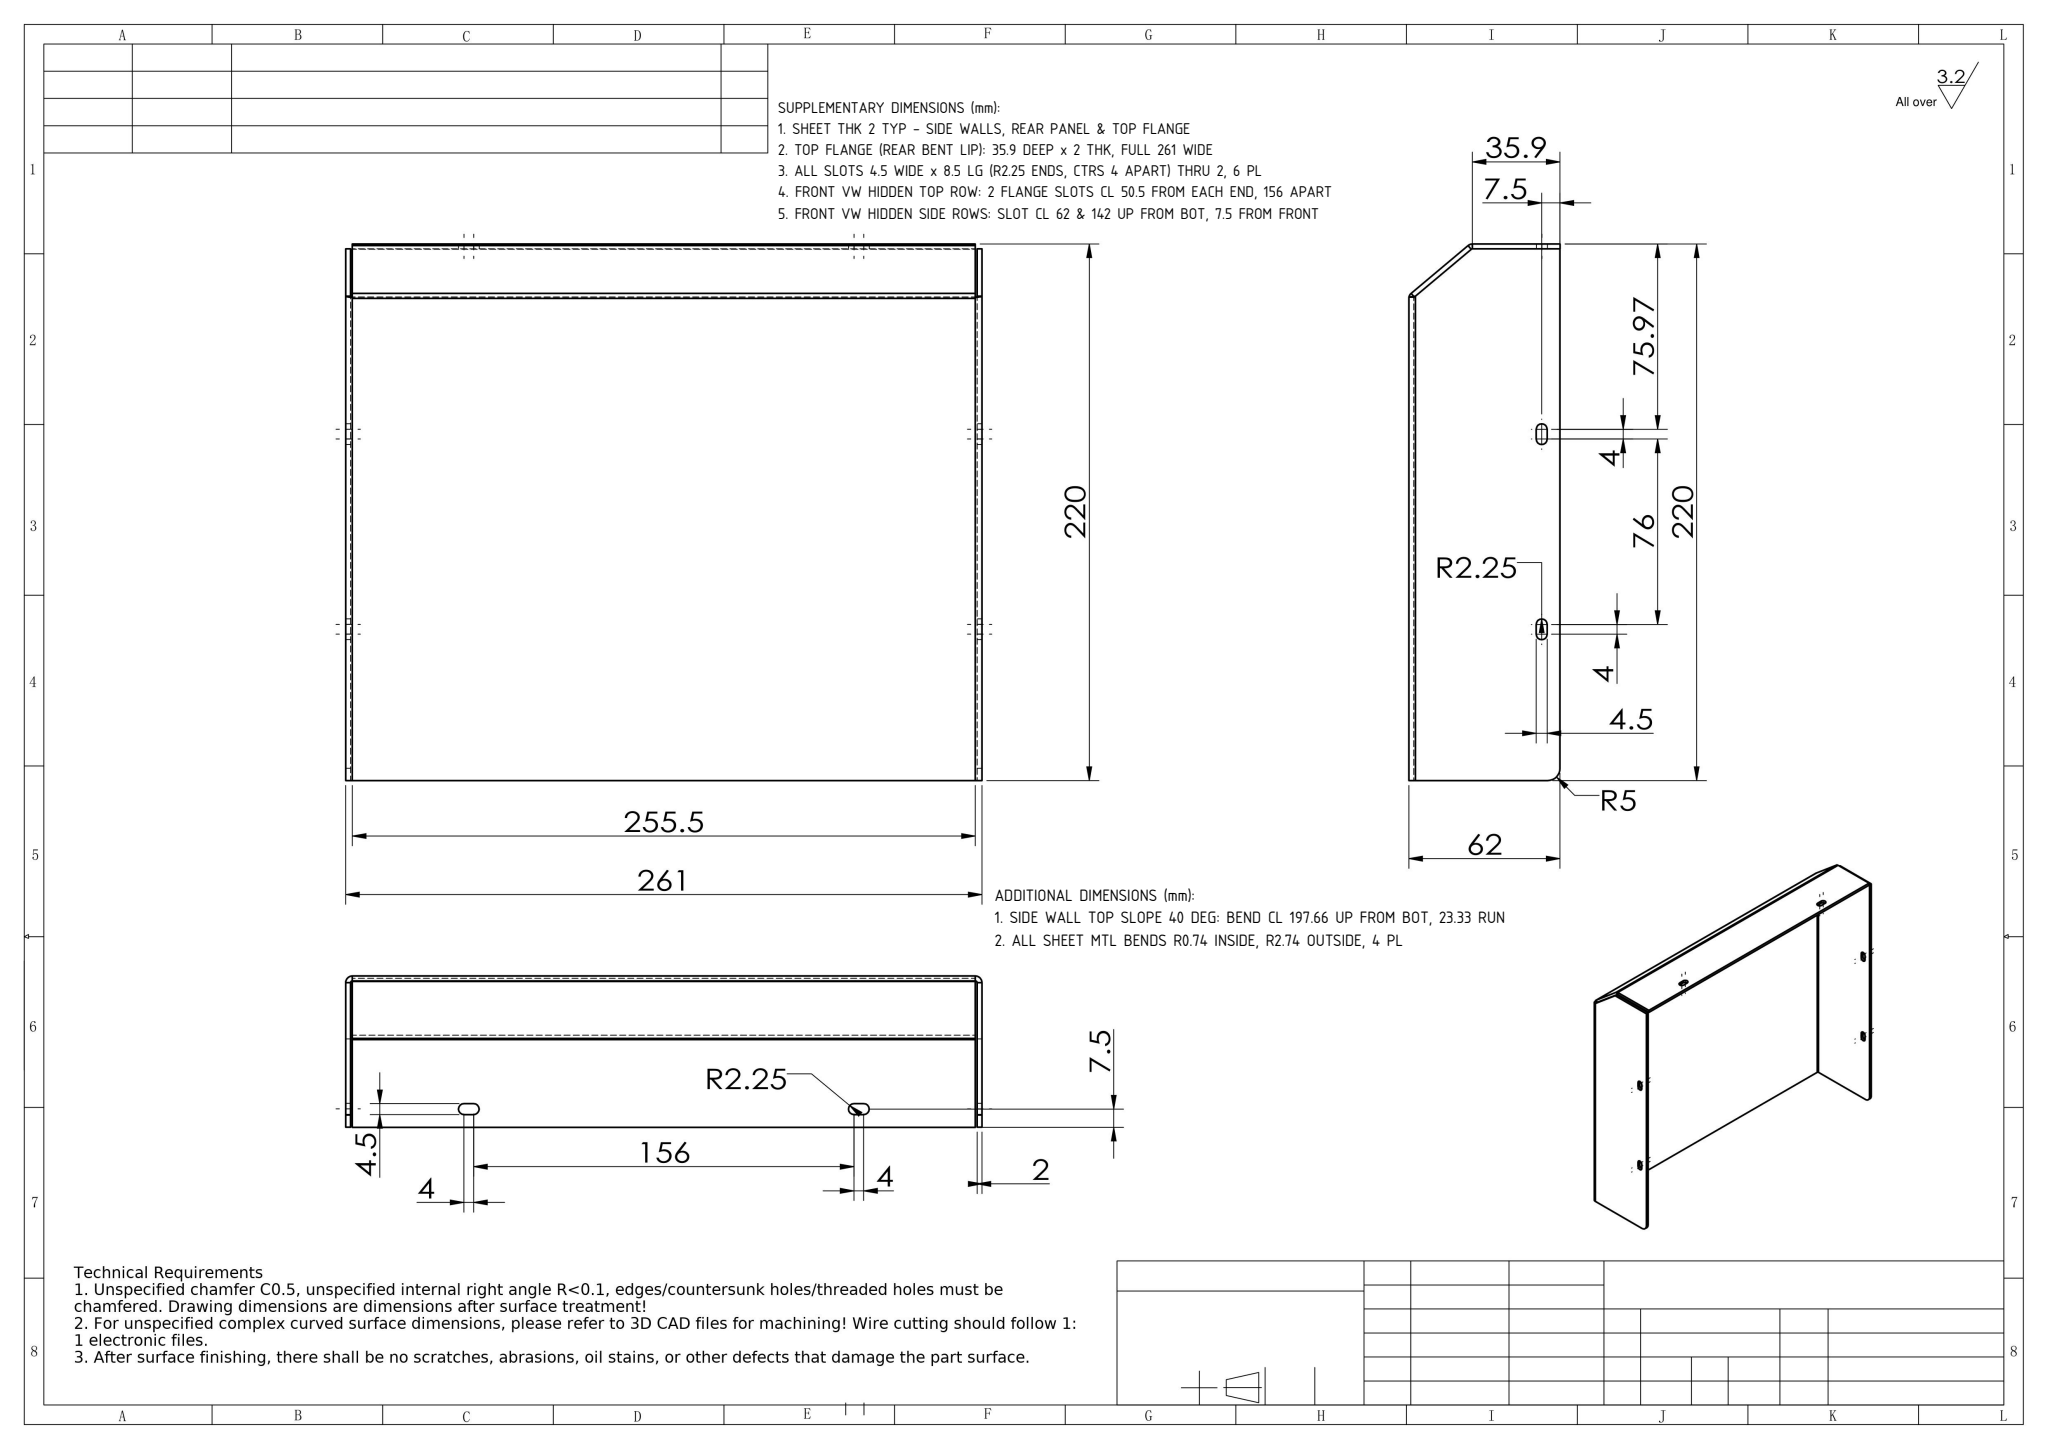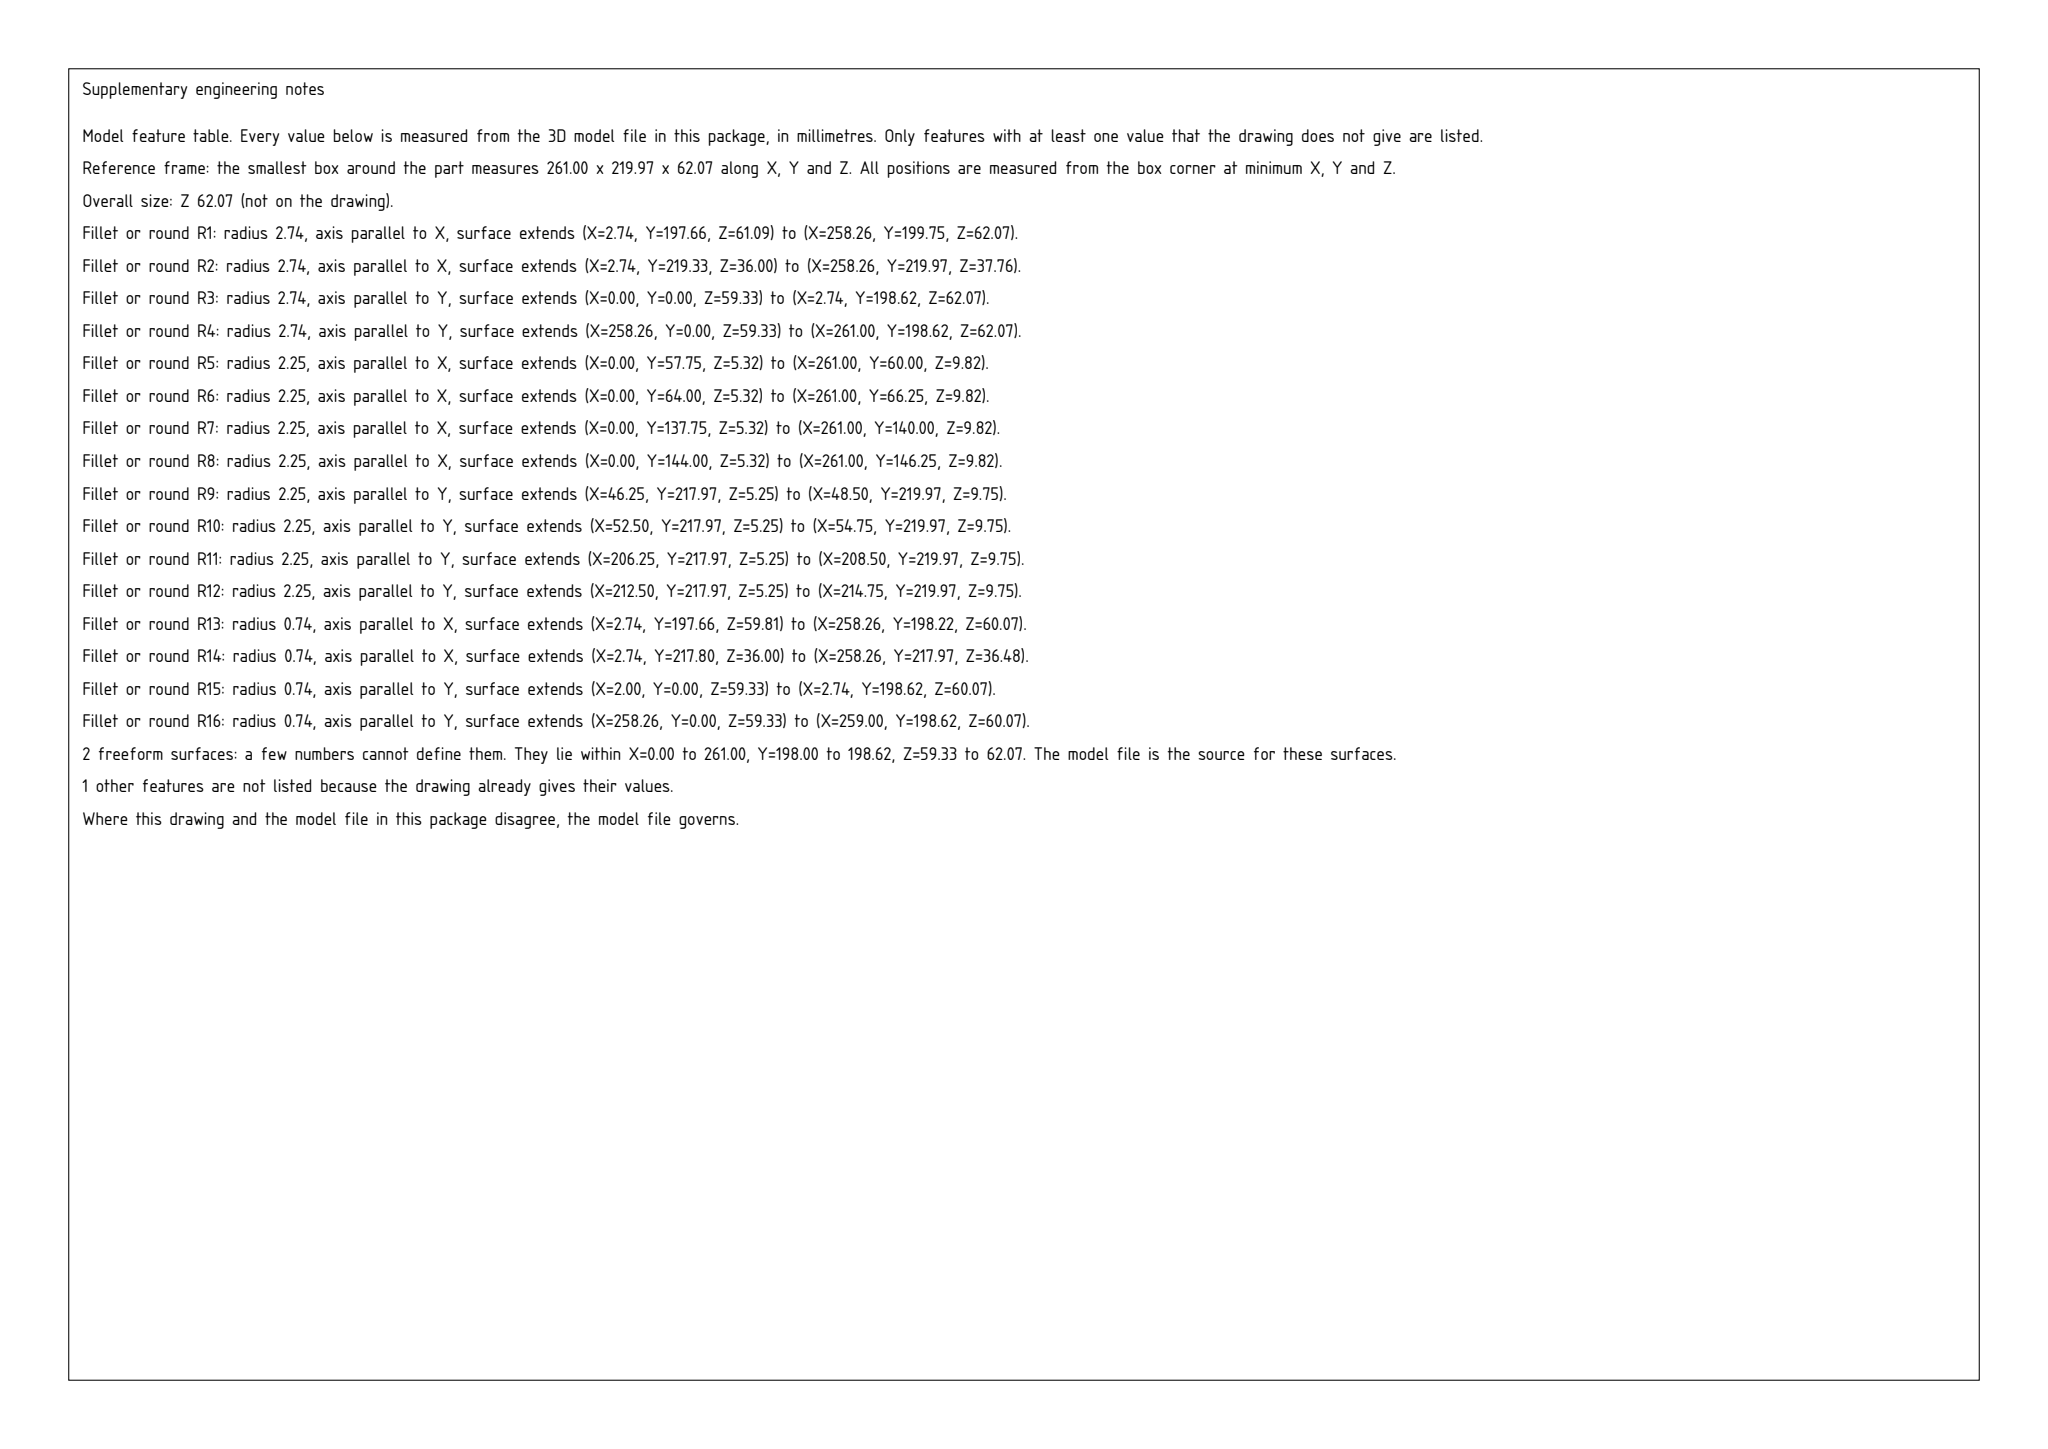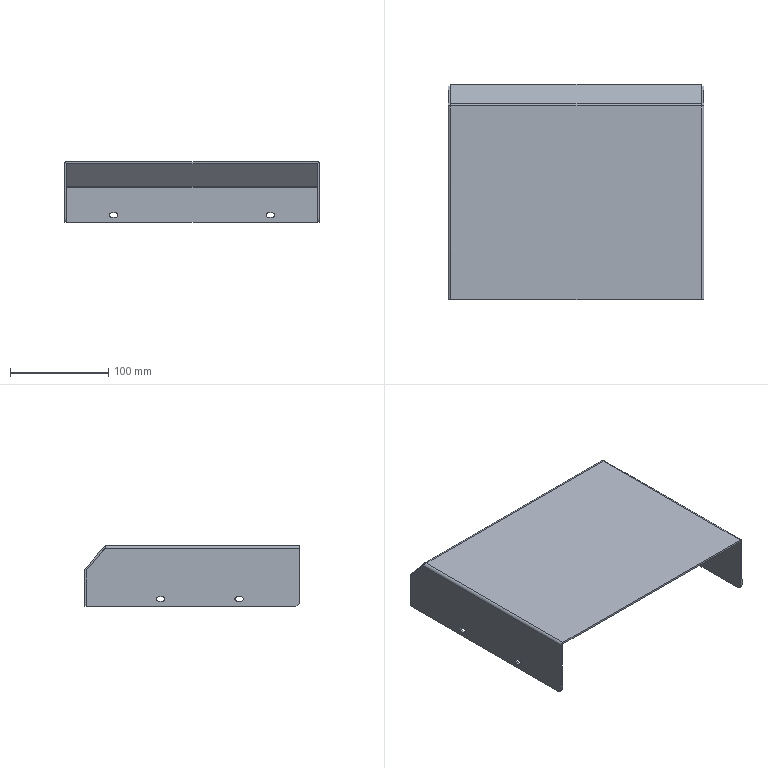Part | SolidWorks | mm | 1 solid | 68 faces | box 261 x 219.97 x 62.07 mm | volume 188889 mm3 | plane 44 | cylinder 22 | spline 2 | commonest cylinder face diameters 4.5 x12 5.473 x4 1.473 x4 10 x2